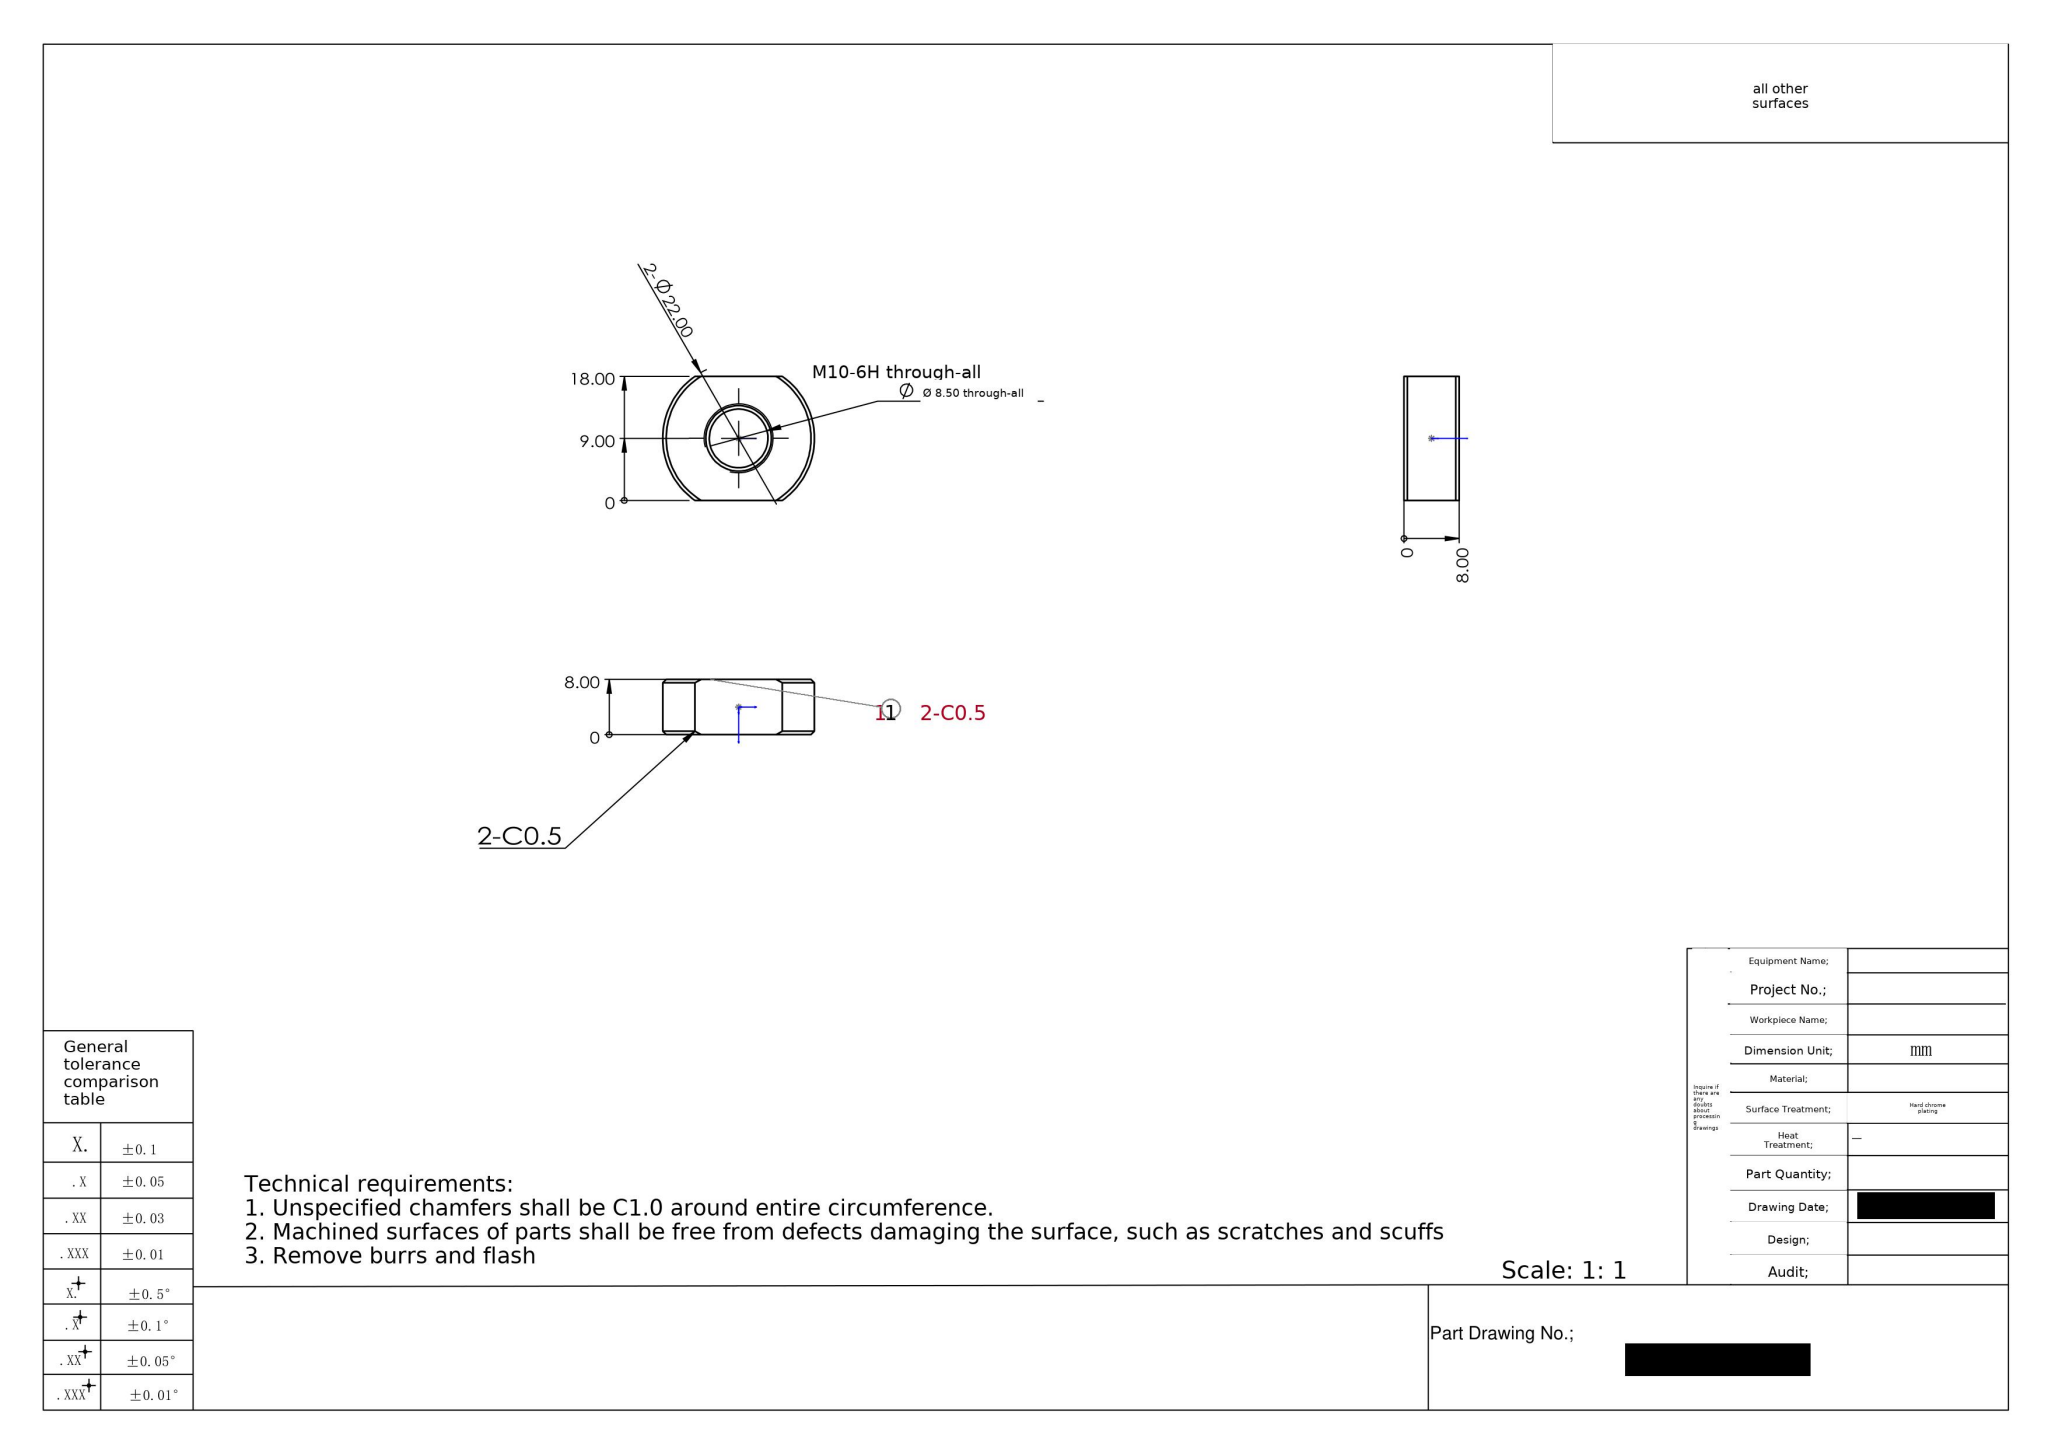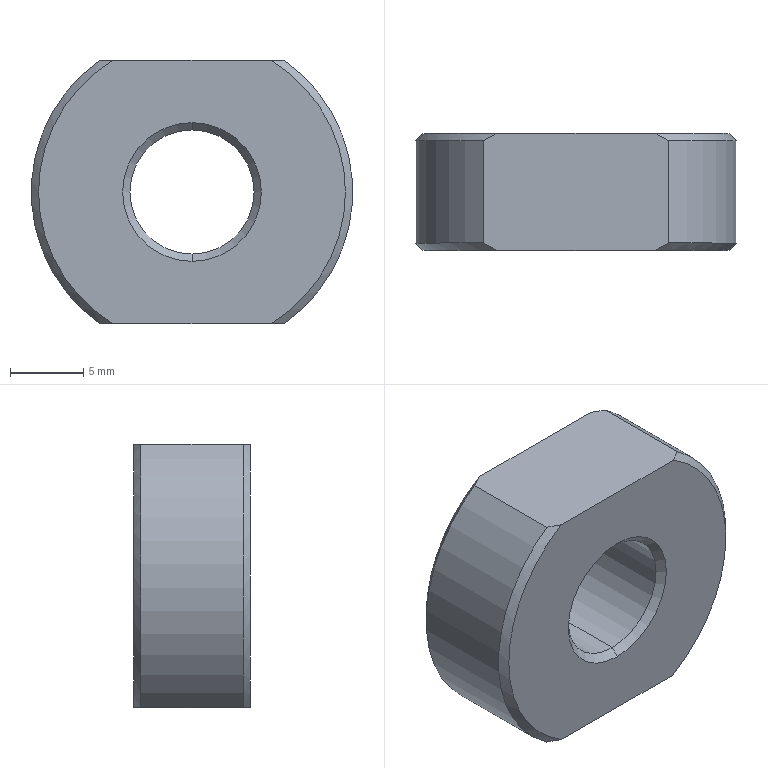Part | SolidWorks | mm | 1 solid | 16 faces | box 22 x 8 x 18 mm | volume 2294 mm3 | cone 8 | cylinder 4 | plane 4 | commonest cylinder face diameters 8.5 x2 22 x2
build123d program:
from build123d import *

# Parameters (mm, degrees)
SKETCH1_W          = 11
SKETCH1_H          = 8
M10X1_5_D          = 8.5
CHAMFER1_SIZE      = 0.5
CUT_EXTRUDE1_DEPTH = 18.493


with BuildPart() as part:
    # Sketch1 → Revolve1 (revolve)
    with BuildSketch(Plane.XY, mode=Mode.PRIVATE) as revolve1_sk:
        with Locations((5.5, 0)):
            Rectangle(SKETCH1_W, SKETCH1_H)
    revolve(revolve1_sk.sketch.rotate(Axis((0, 0, 0), (0, 1, 0)), 90), axis=Axis((0, 0, 0), (0, 1, 0)))

    # M10X1.5 (through all)
    with Locations(Plane(origin=(0, 4, 0), x_dir=(1, 0, 0), z_dir=(0, 1, 0))):
        with Locations((0, 0)):
            Hole(M10X1_5_D / 2)

    # Chamfer1
    chamfer1_edges = [part.edges().sort_by_distance(p)[0] for p in [
        (4.25, 4, 0),
        (4.25, -4, 0),
        (0, -4, 11),
        (0, 4, 11),
    ]]
    chamfer(chamfer1_edges, length=CHAMFER1_SIZE)

    # Sketch5 → Cut-Extrude1 (cut, through all)
    with BuildSketch(Plane(origin=(0, 4, 0), x_dir=(1, 0, 0), z_dir=(0, 1, 0))):
        with BuildLine():
            Line((-6.325, 9), (6.325, 9))
            ThreePointArc((6.325, 9), (0, 11), (-6.325, 9))
        make_face()
        with BuildLine():
            Line((-6.325, -9), (6.325, -9))
            ThreePointArc((6.325, -9), (0, -11), (-6.325, -9))
        make_face()
    extrude(amount=-CUT_EXTRUDE1_DEPTH, mode=Mode.SUBTRACT)


solid = part.part
STEP:
#1=CARTESIAN_POINT('',(0.,3.5,-4.25));
#2=VERTEX_POINT('',#1);
#3=CARTESIAN_POINT('',(0.,3.5,4.25));
#4=VERTEX_POINT('',#3);
#5=CARTESIAN_POINT('',(0.,3.5,0.));
#6=DIRECTION('',(0.,1.,0.));
#7=DIRECTION('',(0.,0.,1.));
#8=AXIS2_PLACEMENT_3D('',#5,#6,#7);
#9=CIRCLE('',#8,4.25);
#10=EDGE_CURVE('',#2,#4,#9,.T.);
#11=ORIENTED_EDGE('',*,*,#10,.F.);
#12=CARTESIAN_POINT('',(0.,4.,-4.75));
#13=VERTEX_POINT('',#12);
#14=CARTESIAN_POINT('',(0.,3.5,-4.25));
#15=DIRECTION('',(0.,0.7071,-0.7071));
#16=VECTOR('',#15,1000.);
#17=LINE('',#14,#16);
#18=EDGE_CURVE('',#2,#13,#17,.T.);
#19=ORIENTED_EDGE('',*,*,#18,.T.);
#20=CARTESIAN_POINT('',(0.,4.,4.75));
#21=VERTEX_POINT('',#20);
#22=CARTESIAN_POINT('',(0.,4.,0.));
#23=DIRECTION('',(0.,-1.,0.));
#24=DIRECTION('',(0.,0.,1.));
#25=AXIS2_PLACEMENT_3D('',#22,#23,#24);
#26=CIRCLE('',#25,4.75);
#27=EDGE_CURVE('',#21,#13,#26,.T.);
#28=ORIENTED_EDGE('',*,*,#27,.F.);
#29=CARTESIAN_POINT('',(0.,3.5,4.25));
#30=DIRECTION('',(0.,0.7071,0.7071));
#31=VECTOR('',#30,1000.);
#32=LINE('',#29,#31);
#33=EDGE_CURVE('',#4,#21,#32,.T.);
#34=ORIENTED_EDGE('',*,*,#33,.F.);
#35=EDGE_LOOP('',(#11,#19,#28,#34));
#36=FACE_OUTER_BOUND('',#35,.T.);
#37=CARTESIAN_POINT('',(0.,3.5,0.));
#38=DIRECTION('',(0.,1.,0.));
#39=DIRECTION('',(0.,0.,1.));
#40=AXIS2_PLACEMENT_3D('',#37,#38,#39);
#41=CONICAL_SURFACE('',#40,4.25,0.7854);
#42=ADVANCED_FACE('',(#36),#41,.F.);
#43=CARTESIAN_POINT('',(0.,-3.5,4.25));
#44=VERTEX_POINT('',#43);
#45=CARTESIAN_POINT('',(0.,-3.5,-4.25));
#46=VERTEX_POINT('',#45);
#47=CARTESIAN_POINT('',(0.,-3.5,0.));
#48=DIRECTION('',(0.,-1.,0.));
#49=DIRECTION('',(0.,0.,-1.));
#50=AXIS2_PLACEMENT_3D('',#47,#48,#49);
#51=CIRCLE('',#50,4.25);
#52=EDGE_CURVE('',#44,#46,#51,.T.);
#53=ORIENTED_EDGE('',*,*,#52,.F.);
#54=CARTESIAN_POINT('',(0.,-4.,4.75));
#55=VERTEX_POINT('',#54);
#56=CARTESIAN_POINT('',(0.,-4.,4.75));
#57=DIRECTION('',(0.,-0.7071,0.7071));
#58=VECTOR('',#57,1000.);
#59=LINE('',#56,#58);
#60=EDGE_CURVE('',#44,#55,#59,.T.);
#61=ORIENTED_EDGE('',*,*,#60,.T.);
#62=CARTESIAN_POINT('',(0.,-4.,-4.75));
#63=VERTEX_POINT('',#62);
#64=CARTESIAN_POINT('',(0.,-4.,0.));
#65=DIRECTION('',(0.,1.,0.));
#66=DIRECTION('',(0.,0.,-1.));
#67=AXIS2_PLACEMENT_3D('',#64,#65,#66);
#68=CIRCLE('',#67,4.75);
#69=EDGE_CURVE('',#63,#55,#68,.T.);
#70=ORIENTED_EDGE('',*,*,#69,.F.);
#71=CARTESIAN_POINT('',(0.,-4.,-4.75));
#72=DIRECTION('',(0.,-0.7071,-0.7071));
#73=VECTOR('',#72,1000.);
#74=LINE('',#71,#73);
#75=EDGE_CURVE('',#46,#63,#74,.T.);
#76=ORIENTED_EDGE('',*,*,#75,.F.);
#77=EDGE_LOOP('',(#53,#61,#70,#76));
#78=FACE_OUTER_BOUND('',#77,.T.);
#79=CARTESIAN_POINT('',(0.,-4.,0.));
#80=DIRECTION('',(0.,-1.,0.));
#81=DIRECTION('',(0.,0.,-1.));
#82=AXIS2_PLACEMENT_3D('',#79,#80,#81);
#83=CONICAL_SURFACE('',#82,4.75,0.7854);
#84=ADVANCED_FACE('',(#78),#83,.F.);
#85=ORIENTED_EDGE('',*,*,#52,.T.);
#86=CARTESIAN_POINT('',(0.,4.,-4.25));
#87=DIRECTION('',(0.,1.,0.));
#88=VECTOR('',#87,1000.);
#89=LINE('',#86,#88);
#90=EDGE_CURVE('',#46,#2,#89,.T.);
#91=ORIENTED_EDGE('',*,*,#90,.T.);
#92=ORIENTED_EDGE('',*,*,#10,.T.);
#93=CARTESIAN_POINT('',(0.,4.,4.25));
#94=DIRECTION('',(0.,1.,0.));
#95=VECTOR('',#94,1000.);
#96=LINE('',#93,#95);
#97=EDGE_CURVE('',#44,#4,#96,.T.);
#98=ORIENTED_EDGE('',*,*,#97,.F.);
#99=EDGE_LOOP('',(#85,#91,#92,#98));
#100=FACE_OUTER_BOUND('',#99,.T.);
#101=CARTESIAN_POINT('',(0.,4.,0.));
#102=DIRECTION('',(0.,1.,0.));
#103=DIRECTION('',(0.,0.,1.));
#104=AXIS2_PLACEMENT_3D('',#101,#102,#103);
#105=CYLINDRICAL_SURFACE('',#104,4.25);
#106=ADVANCED_FACE('',(#100),#105,.F.);
#107=CARTESIAN_POINT('',(6.325,-3.5,9.));
#108=VERTEX_POINT('',#107);
#109=CARTESIAN_POINT('',(6.325,3.5,9.));
#110=VERTEX_POINT('',#109);
#111=CARTESIAN_POINT('',(6.325,-4.,9.));
#112=DIRECTION('',(0.,1.,0.));
#113=VECTOR('',#112,1000.);
#114=LINE('',#111,#113);
#115=EDGE_CURVE('',#108,#110,#114,.T.);
#116=ORIENTED_EDGE('',*,*,#115,.F.);
#117=CARTESIAN_POINT('',(6.325,-3.5,-9.));
#118=VERTEX_POINT('',#117);
#119=CARTESIAN_POINT('',(0.,-3.5,0.));
#120=DIRECTION('',(0.,1.,0.));
#121=DIRECTION('',(0.,0.,-1.));
#122=AXIS2_PLACEMENT_3D('',#119,#120,#121);
#123=CIRCLE('',#122,11.);
#124=EDGE_CURVE('',#108,#118,#123,.T.);
#125=ORIENTED_EDGE('',*,*,#124,.T.);
#126=CARTESIAN_POINT('',(6.325,3.5,-9.));
#127=VERTEX_POINT('',#126);
#128=CARTESIAN_POINT('',(6.325,-4.,-9.));
#129=DIRECTION('',(0.,1.,0.));
#130=VECTOR('',#129,1000.);
#131=LINE('',#128,#130);
#132=EDGE_CURVE('',#118,#127,#131,.T.);
#133=ORIENTED_EDGE('',*,*,#132,.T.);
#134=CARTESIAN_POINT('',(0.,3.5,0.));
#135=DIRECTION('',(0.,-1.,0.));
#136=DIRECTION('',(0.,0.,1.));
#137=AXIS2_PLACEMENT_3D('',#134,#135,#136);
#138=CIRCLE('',#137,11.);
#139=EDGE_CURVE('',#127,#110,#138,.T.);
#140=ORIENTED_EDGE('',*,*,#139,.T.);
#141=EDGE_LOOP('',(#116,#125,#133,#140));
#142=FACE_OUTER_BOUND('',#141,.T.);
#143=CARTESIAN_POINT('',(0.,0.,0.));
#144=DIRECTION('',(0.,-1.,0.));
#145=DIRECTION('',(0.,0.,-1.));
#146=AXIS2_PLACEMENT_3D('',#143,#144,#145);
#147=CYLINDRICAL_SURFACE('',#146,11.);
#148=ADVANCED_FACE('',(#142),#147,.T.);
#149=CARTESIAN_POINT('',(-6.325,-3.5,9.));
#150=VERTEX_POINT('',#149);
#151=CARTESIAN_POINT('',(-5.408,-4.,9.));
#152=VERTEX_POINT('',#151);
#153=CARTESIAN_POINT('',(-6.325,-3.5,9.));
#154=CARTESIAN_POINT('',(-6.023,-3.674,9.));
#155=CARTESIAN_POINT('',(-5.717,-3.841,9.));
#156=CARTESIAN_POINT('',(-5.408,-4.,9.));
#157=B_SPLINE_CURVE_WITH_KNOTS('',3,(#153,#154,#155,#156),.UNSPECIFIED.,.F.,.F.,(4,4),(0.009438,0.01049),.UNSPECIFIED.);
#158=EDGE_CURVE('',#150,#152,#157,.T.);
#159=ORIENTED_EDGE('',*,*,#158,.F.);
#160=CARTESIAN_POINT('',(-6.325,-3.5,-9.));
#161=VERTEX_POINT('',#160);
#162=CARTESIAN_POINT('',(0.,-3.5,0.));
#163=DIRECTION('',(0.,1.,0.));
#164=DIRECTION('',(0.,0.,-1.));
#165=AXIS2_PLACEMENT_3D('',#162,#163,#164);
#166=CIRCLE('',#165,11.);
#167=EDGE_CURVE('',#161,#150,#166,.T.);
#168=ORIENTED_EDGE('',*,*,#167,.F.);
#169=CARTESIAN_POINT('',(-5.408,-4.,-9.));
#170=VERTEX_POINT('',#169);
#171=CARTESIAN_POINT('',(-5.408,-4.,-9.));
#172=CARTESIAN_POINT('',(-5.718,-3.841,-9.));
#173=CARTESIAN_POINT('',(-6.024,-3.673,-9.));
#174=CARTESIAN_POINT('',(-6.325,-3.5,-9.));
#175=B_SPLINE_CURVE_WITH_KNOTS('',3,(#171,#172,#173,#174),.UNSPECIFIED.,.F.,.F.,(4,4),(0.02178,0.02281),.UNSPECIFIED.);
#176=EDGE_CURVE('',#170,#161,#175,.T.);
#177=ORIENTED_EDGE('',*,*,#176,.F.);
#178=CARTESIAN_POINT('',(0.,-4.,0.));
#179=DIRECTION('',(0.,-1.,0.));
#180=DIRECTION('',(0.,0.,-1.));
#181=AXIS2_PLACEMENT_3D('',#178,#179,#180);
#182=CIRCLE('',#181,10.5);
#183=EDGE_CURVE('',#152,#170,#182,.T.);
#184=ORIENTED_EDGE('',*,*,#183,.F.);
#185=EDGE_LOOP('',(#159,#168,#177,#184));
#186=FACE_OUTER_BOUND('',#185,.T.);
#187=CARTESIAN_POINT('',(0.,-4.,0.));
#188=DIRECTION('',(0.,1.,0.));
#189=DIRECTION('',(0.,0.,1.));
#190=AXIS2_PLACEMENT_3D('',#187,#188,#189);
#191=CONICAL_SURFACE('',#190,10.5,0.7854);
#192=ADVANCED_FACE('',(#186),#191,.T.);
#193=CARTESIAN_POINT('',(5.408,4.,9.));
#194=VERTEX_POINT('',#193);
#195=CARTESIAN_POINT('',(6.325,3.5,9.));
#196=CARTESIAN_POINT('',(6.023,3.674,9.));
#197=CARTESIAN_POINT('',(5.717,3.841,9.));
#198=CARTESIAN_POINT('',(5.408,4.,9.));
#199=B_SPLINE_CURVE_WITH_KNOTS('',3,(#195,#196,#197,#198),.UNSPECIFIED.,.F.,.F.,(4,4),(0.009438,0.01049),.UNSPECIFIED.);
#200=EDGE_CURVE('',#110,#194,#199,.T.);
#201=ORIENTED_EDGE('',*,*,#200,.F.);
#202=ORIENTED_EDGE('',*,*,#139,.F.);
#203=CARTESIAN_POINT('',(5.408,4.,-9.));
#204=VERTEX_POINT('',#203);
#205=CARTESIAN_POINT('',(5.408,4.,-9.));
#206=CARTESIAN_POINT('',(5.718,3.841,-9.));
#207=CARTESIAN_POINT('',(6.024,3.673,-9.));
#208=CARTESIAN_POINT('',(6.325,3.5,-9.));
#209=B_SPLINE_CURVE_WITH_KNOTS('',3,(#205,#206,#207,#208),.UNSPECIFIED.,.F.,.F.,(4,4),(0.02178,0.02281),.UNSPECIFIED.);
#210=EDGE_CURVE('',#204,#127,#209,.T.);
#211=ORIENTED_EDGE('',*,*,#210,.F.);
#212=CARTESIAN_POINT('',(0.,4.,0.));
#213=DIRECTION('',(0.,1.,0.));
#214=DIRECTION('',(0.,0.,1.));
#215=AXIS2_PLACEMENT_3D('',#212,#213,#214);
#216=CIRCLE('',#215,10.5);
#217=EDGE_CURVE('',#194,#204,#216,.T.);
#218=ORIENTED_EDGE('',*,*,#217,.F.);
#219=EDGE_LOOP('',(#201,#202,#211,#218));
#220=FACE_OUTER_BOUND('',#219,.T.);
#221=CARTESIAN_POINT('',(0.,3.5,0.));
#222=DIRECTION('',(0.,-1.,0.));
#223=DIRECTION('',(0.,0.,-1.));
#224=AXIS2_PLACEMENT_3D('',#221,#222,#223);
#225=CONICAL_SURFACE('',#224,11.,0.7854);
#226=ADVANCED_FACE('',(#220),#225,.T.);
#227=CARTESIAN_POINT('',(-5.408,4.,9.));
#228=VERTEX_POINT('',#227);
#229=CARTESIAN_POINT('',(-6.325,4.,9.));
#230=DIRECTION('',(-1.,0.,0.));
#231=VECTOR('',#230,1000.);
#232=LINE('',#229,#231);
#233=EDGE_CURVE('',#194,#228,#232,.T.);
#234=ORIENTED_EDGE('',*,*,#233,.F.);
#235=ORIENTED_EDGE('',*,*,#217,.T.);
#236=CARTESIAN_POINT('',(-5.408,4.,-9.));
#237=VERTEX_POINT('',#236);
#238=CARTESIAN_POINT('',(-6.325,4.,-9.));
#239=DIRECTION('',(1.,0.,0.));
#240=VECTOR('',#239,1000.);
#241=LINE('',#238,#240);
#242=EDGE_CURVE('',#237,#204,#241,.T.);
#243=ORIENTED_EDGE('',*,*,#242,.F.);
#244=CARTESIAN_POINT('',(0.,4.,0.));
#245=DIRECTION('',(0.,1.,0.));
#246=DIRECTION('',(0.,0.,1.));
#247=AXIS2_PLACEMENT_3D('',#244,#245,#246);
#248=CIRCLE('',#247,10.5);
#249=EDGE_CURVE('',#237,#228,#248,.T.);
#250=ORIENTED_EDGE('',*,*,#249,.T.);
#251=EDGE_LOOP('',(#234,#235,#243,#250));
#252=FACE_OUTER_BOUND('',#251,.T.);
#253=ORIENTED_EDGE('',*,*,#27,.T.);
#254=CARTESIAN_POINT('',(0.,4.,0.));
#255=DIRECTION('',(0.,-1.,0.));
#256=DIRECTION('',(0.,0.,1.));
#257=AXIS2_PLACEMENT_3D('',#254,#255,#256);
#258=CIRCLE('',#257,4.75);
#259=EDGE_CURVE('',#13,#21,#258,.T.);
#260=ORIENTED_EDGE('',*,*,#259,.T.);
#261=EDGE_LOOP('',(#253,#260));
#262=FACE_BOUND('',#261,.T.);
#263=CARTESIAN_POINT('',(0.,4.,0.));
#264=DIRECTION('',(0.,1.,0.));
#265=DIRECTION('',(0.,0.,1.));
#266=AXIS2_PLACEMENT_3D('',#263,#264,#265);
#267=PLANE('',#266);
#268=ADVANCED_FACE('',(#252,#262),#267,.T.);
#269=CARTESIAN_POINT('',(-6.325,3.5,9.));
#270=VERTEX_POINT('',#269);
#271=CARTESIAN_POINT('',(-6.325,-4.,9.));
#272=DIRECTION('',(0.,1.,0.));
#273=VECTOR('',#272,1000.);
#274=LINE('',#271,#273);
#275=EDGE_CURVE('',#150,#270,#274,.T.);
#276=ORIENTED_EDGE('',*,*,#275,.T.);
#277=CARTESIAN_POINT('',(-6.325,3.5,-9.));
#278=VERTEX_POINT('',#277);
#279=CARTESIAN_POINT('',(0.,3.5,0.));
#280=DIRECTION('',(0.,-1.,0.));
#281=DIRECTION('',(0.,0.,1.));
#282=AXIS2_PLACEMENT_3D('',#279,#280,#281);
#283=CIRCLE('',#282,11.);
#284=EDGE_CURVE('',#270,#278,#283,.T.);
#285=ORIENTED_EDGE('',*,*,#284,.T.);
#286=CARTESIAN_POINT('',(-6.325,-4.,-9.));
#287=DIRECTION('',(0.,1.,0.));
#288=VECTOR('',#287,1000.);
#289=LINE('',#286,#288);
#290=EDGE_CURVE('',#161,#278,#289,.T.);
#291=ORIENTED_EDGE('',*,*,#290,.F.);
#292=ORIENTED_EDGE('',*,*,#167,.T.);
#293=EDGE_LOOP('',(#276,#285,#291,#292));
#294=FACE_OUTER_BOUND('',#293,.T.);
#295=CARTESIAN_POINT('',(0.,0.,0.));
#296=DIRECTION('',(0.,-1.,0.));
#297=DIRECTION('',(0.,0.,-1.));
#298=AXIS2_PLACEMENT_3D('',#295,#296,#297);
#299=CYLINDRICAL_SURFACE('',#298,11.);
#300=ADVANCED_FACE('',(#294),#299,.T.);
#301=CARTESIAN_POINT('',(5.408,-4.,9.));
#302=VERTEX_POINT('',#301);
#303=CARTESIAN_POINT('',(-6.325,-4.,9.));
#304=DIRECTION('',(-1.,0.,0.));
#305=VECTOR('',#304,1000.);
#306=LINE('',#303,#305);
#307=EDGE_CURVE('',#302,#152,#306,.T.);
#308=ORIENTED_EDGE('',*,*,#307,.T.);
#309=ORIENTED_EDGE('',*,*,#183,.T.);
#310=CARTESIAN_POINT('',(5.408,-4.,-9.));
#311=VERTEX_POINT('',#310);
#312=CARTESIAN_POINT('',(-6.325,-4.,-9.));
#313=DIRECTION('',(1.,0.,0.));
#314=VECTOR('',#313,1000.);
#315=LINE('',#312,#314);
#316=EDGE_CURVE('',#170,#311,#315,.T.);
#317=ORIENTED_EDGE('',*,*,#316,.T.);
#318=CARTESIAN_POINT('',(0.,-4.,0.));
#319=DIRECTION('',(0.,-1.,0.));
#320=DIRECTION('',(0.,0.,-1.));
#321=AXIS2_PLACEMENT_3D('',#318,#319,#320);
#322=CIRCLE('',#321,10.5);
#323=EDGE_CURVE('',#311,#302,#322,.T.);
#324=ORIENTED_EDGE('',*,*,#323,.T.);
#325=EDGE_LOOP('',(#308,#309,#317,#324));
#326=FACE_OUTER_BOUND('',#325,.T.);
#327=ORIENTED_EDGE('',*,*,#69,.T.);
#328=CARTESIAN_POINT('',(0.,-4.,0.));
#329=DIRECTION('',(0.,1.,0.));
#330=DIRECTION('',(0.,0.,-1.));
#331=AXIS2_PLACEMENT_3D('',#328,#329,#330);
#332=CIRCLE('',#331,4.75);
#333=EDGE_CURVE('',#55,#63,#332,.T.);
#334=ORIENTED_EDGE('',*,*,#333,.T.);
#335=EDGE_LOOP('',(#327,#334));
#336=FACE_BOUND('',#335,.T.);
#337=CARTESIAN_POINT('',(11.,-4.,0.));
#338=DIRECTION('',(0.,-1.,0.));
#339=DIRECTION('',(0.,0.,-1.));
#340=AXIS2_PLACEMENT_3D('',#337,#338,#339);
#341=PLANE('',#340);
#342=ADVANCED_FACE('',(#326,#336),#341,.T.);
#343=ORIENTED_EDGE('',*,*,#90,.F.);
#344=CARTESIAN_POINT('',(0.,-3.5,0.));
#345=DIRECTION('',(0.,-1.,0.));
#346=DIRECTION('',(0.,0.,-1.));
#347=AXIS2_PLACEMENT_3D('',#344,#345,#346);
#348=CIRCLE('',#347,4.25);
#349=EDGE_CURVE('',#46,#44,#348,.T.);
#350=ORIENTED_EDGE('',*,*,#349,.T.);
#351=ORIENTED_EDGE('',*,*,#97,.T.);
#352=CARTESIAN_POINT('',(0.,3.5,0.));
#353=DIRECTION('',(0.,1.,0.));
#354=DIRECTION('',(0.,0.,1.));
#355=AXIS2_PLACEMENT_3D('',#352,#353,#354);
#356=CIRCLE('',#355,4.25);
#357=EDGE_CURVE('',#4,#2,#356,.T.);
#358=ORIENTED_EDGE('',*,*,#357,.T.);
#359=EDGE_LOOP('',(#343,#350,#351,#358));
#360=FACE_OUTER_BOUND('',#359,.T.);
#361=CARTESIAN_POINT('',(0.,4.,0.));
#362=DIRECTION('',(0.,1.,0.));
#363=DIRECTION('',(0.,0.,1.));
#364=AXIS2_PLACEMENT_3D('',#361,#362,#363);
#365=CYLINDRICAL_SURFACE('',#364,4.25);
#366=ADVANCED_FACE('',(#360),#365,.F.);
#367=ORIENTED_EDGE('',*,*,#60,.F.);
#368=ORIENTED_EDGE('',*,*,#349,.F.);
#369=ORIENTED_EDGE('',*,*,#75,.T.);
#370=ORIENTED_EDGE('',*,*,#333,.F.);
#371=EDGE_LOOP('',(#367,#368,#369,#370));
#372=FACE_OUTER_BOUND('',#371,.T.);
#373=CARTESIAN_POINT('',(0.,-4.,0.));
#374=DIRECTION('',(0.,-1.,0.));
#375=DIRECTION('',(0.,0.,-1.));
#376=AXIS2_PLACEMENT_3D('',#373,#374,#375);
#377=CONICAL_SURFACE('',#376,4.75,0.7854);
#378=ADVANCED_FACE('',(#372),#377,.F.);
#379=ORIENTED_EDGE('',*,*,#18,.F.);
#380=ORIENTED_EDGE('',*,*,#357,.F.);
#381=ORIENTED_EDGE('',*,*,#33,.T.);
#382=ORIENTED_EDGE('',*,*,#259,.F.);
#383=EDGE_LOOP('',(#379,#380,#381,#382));
#384=FACE_OUTER_BOUND('',#383,.T.);
#385=CARTESIAN_POINT('',(0.,3.5,0.));
#386=DIRECTION('',(0.,1.,0.));
#387=DIRECTION('',(0.,0.,1.));
#388=AXIS2_PLACEMENT_3D('',#385,#386,#387);
#389=CONICAL_SURFACE('',#388,4.25,0.7854);
#390=ADVANCED_FACE('',(#384),#389,.F.);
#391=CARTESIAN_POINT('',(5.408,-4.,9.));
#392=CARTESIAN_POINT('',(5.718,-3.841,9.));
#393=CARTESIAN_POINT('',(6.024,-3.673,9.));
#394=CARTESIAN_POINT('',(6.325,-3.5,9.));
#395=B_SPLINE_CURVE_WITH_KNOTS('',3,(#391,#392,#393,#394),.UNSPECIFIED.,.F.,.F.,(4,4),(0.02178,0.02281),.UNSPECIFIED.);
#396=EDGE_CURVE('',#302,#108,#395,.T.);
#397=ORIENTED_EDGE('',*,*,#396,.F.);
#398=ORIENTED_EDGE('',*,*,#323,.F.);
#399=CARTESIAN_POINT('',(6.325,-3.5,-9.));
#400=CARTESIAN_POINT('',(6.023,-3.674,-9.));
#401=CARTESIAN_POINT('',(5.717,-3.841,-9.));
#402=CARTESIAN_POINT('',(5.408,-4.,-9.));
#403=B_SPLINE_CURVE_WITH_KNOTS('',3,(#399,#400,#401,#402),.UNSPECIFIED.,.F.,.F.,(4,4),(0.009438,0.01049),.UNSPECIFIED.);
#404=EDGE_CURVE('',#118,#311,#403,.T.);
#405=ORIENTED_EDGE('',*,*,#404,.F.);
#406=ORIENTED_EDGE('',*,*,#124,.F.);
#407=EDGE_LOOP('',(#397,#398,#405,#406));
#408=FACE_OUTER_BOUND('',#407,.T.);
#409=CARTESIAN_POINT('',(0.,-4.,0.));
#410=DIRECTION('',(0.,1.,0.));
#411=DIRECTION('',(0.,0.,1.));
#412=AXIS2_PLACEMENT_3D('',#409,#410,#411);
#413=CONICAL_SURFACE('',#412,10.5,0.7854);
#414=ADVANCED_FACE('',(#408),#413,.T.);
#415=CARTESIAN_POINT('',(-5.408,4.,9.));
#416=CARTESIAN_POINT('',(-5.718,3.841,9.));
#417=CARTESIAN_POINT('',(-6.024,3.673,9.));
#418=CARTESIAN_POINT('',(-6.325,3.5,9.));
#419=B_SPLINE_CURVE_WITH_KNOTS('',3,(#415,#416,#417,#418),.UNSPECIFIED.,.F.,.F.,(4,4),(0.02178,0.02281),.UNSPECIFIED.);
#420=EDGE_CURVE('',#228,#270,#419,.T.);
#421=ORIENTED_EDGE('',*,*,#420,.F.);
#422=ORIENTED_EDGE('',*,*,#249,.F.);
#423=CARTESIAN_POINT('',(-6.325,3.5,-9.));
#424=CARTESIAN_POINT('',(-6.023,3.674,-9.));
#425=CARTESIAN_POINT('',(-5.717,3.841,-9.));
#426=CARTESIAN_POINT('',(-5.408,4.,-9.));
#427=B_SPLINE_CURVE_WITH_KNOTS('',3,(#423,#424,#425,#426),.UNSPECIFIED.,.F.,.F.,(4,4),(0.009438,0.01049),.UNSPECIFIED.);
#428=EDGE_CURVE('',#278,#237,#427,.T.);
#429=ORIENTED_EDGE('',*,*,#428,.F.);
#430=ORIENTED_EDGE('',*,*,#284,.F.);
#431=EDGE_LOOP('',(#421,#422,#429,#430));
#432=FACE_OUTER_BOUND('',#431,.T.);
#433=CARTESIAN_POINT('',(0.,3.5,0.));
#434=DIRECTION('',(0.,-1.,0.));
#435=DIRECTION('',(0.,0.,-1.));
#436=AXIS2_PLACEMENT_3D('',#433,#434,#435);
#437=CONICAL_SURFACE('',#436,11.,0.7854);
#438=ADVANCED_FACE('',(#432),#437,.T.);
#439=ORIENTED_EDGE('',*,*,#404,.T.);
#440=ORIENTED_EDGE('',*,*,#316,.F.);
#441=ORIENTED_EDGE('',*,*,#176,.T.);
#442=ORIENTED_EDGE('',*,*,#290,.T.);
#443=ORIENTED_EDGE('',*,*,#428,.T.);
#444=ORIENTED_EDGE('',*,*,#242,.T.);
#445=ORIENTED_EDGE('',*,*,#210,.T.);
#446=ORIENTED_EDGE('',*,*,#132,.F.);
#447=EDGE_LOOP('',(#439,#440,#441,#442,#443,#444,#445,#446));
#448=FACE_OUTER_BOUND('',#447,.T.);
#449=CARTESIAN_POINT('',(-6.325,-4.,-9.));
#450=DIRECTION('',(0.,0.,1.));
#451=DIRECTION('',(1.,0.,0.));
#452=AXIS2_PLACEMENT_3D('',#449,#450,#451);
#453=PLANE('',#452);
#454=ADVANCED_FACE('',(#448),#453,.F.);
#455=ORIENTED_EDGE('',*,*,#158,.T.);
#456=ORIENTED_EDGE('',*,*,#307,.F.);
#457=ORIENTED_EDGE('',*,*,#396,.T.);
#458=ORIENTED_EDGE('',*,*,#115,.T.);
#459=ORIENTED_EDGE('',*,*,#200,.T.);
#460=ORIENTED_EDGE('',*,*,#233,.T.);
#461=ORIENTED_EDGE('',*,*,#420,.T.);
#462=ORIENTED_EDGE('',*,*,#275,.F.);
#463=EDGE_LOOP('',(#455,#456,#457,#458,#459,#460,#461,#462));
#464=FACE_OUTER_BOUND('',#463,.T.);
#465=CARTESIAN_POINT('',(-6.325,-4.,9.));
#466=DIRECTION('',(0.,0.,-1.));
#467=DIRECTION('',(-1.,0.,0.));
#468=AXIS2_PLACEMENT_3D('',#465,#466,#467);
#469=PLANE('',#468);
#470=ADVANCED_FACE('',(#464),#469,.F.);
#471=CLOSED_SHELL('',(#42,#84,#106,#148,#192,#226,#268,#300,#342,#366,#378,#390,#414,#438,#454,#470));
#472=MANIFOLD_SOLID_BREP('',#471);
#473=CARTESIAN_POINT('',(0.,0.,0.));
#474=DIRECTION('',(0.,0.,1.));
#475=DIRECTION('',(1.,0.,0.));
#476=AXIS2_PLACEMENT_3D('',#473,#474,#475);
#477=(LENGTH_UNIT()NAMED_UNIT(*)SI_UNIT(.MILLI.,.METRE.));
#478=UNCERTAINTY_MEASURE_WITH_UNIT(LENGTH_MEASURE(0.00001),#477,'','');
#479=(NAMED_UNIT(*)PLANE_ANGLE_UNIT()SI_UNIT($,.RADIAN.));
#480=(NAMED_UNIT(*)SI_UNIT($,.STERADIAN.)SOLID_ANGLE_UNIT());
#481=(GEOMETRIC_REPRESENTATION_CONTEXT(3)GLOBAL_UNCERTAINTY_ASSIGNED_CONTEXT((#478))GLOBAL_UNIT_ASSIGNED_CONTEXT((#477,#479,#480))REPRESENTATION_CONTEXT('',''));
#482=ADVANCED_BREP_SHAPE_REPRESENTATION('',(#472,#476),#481);